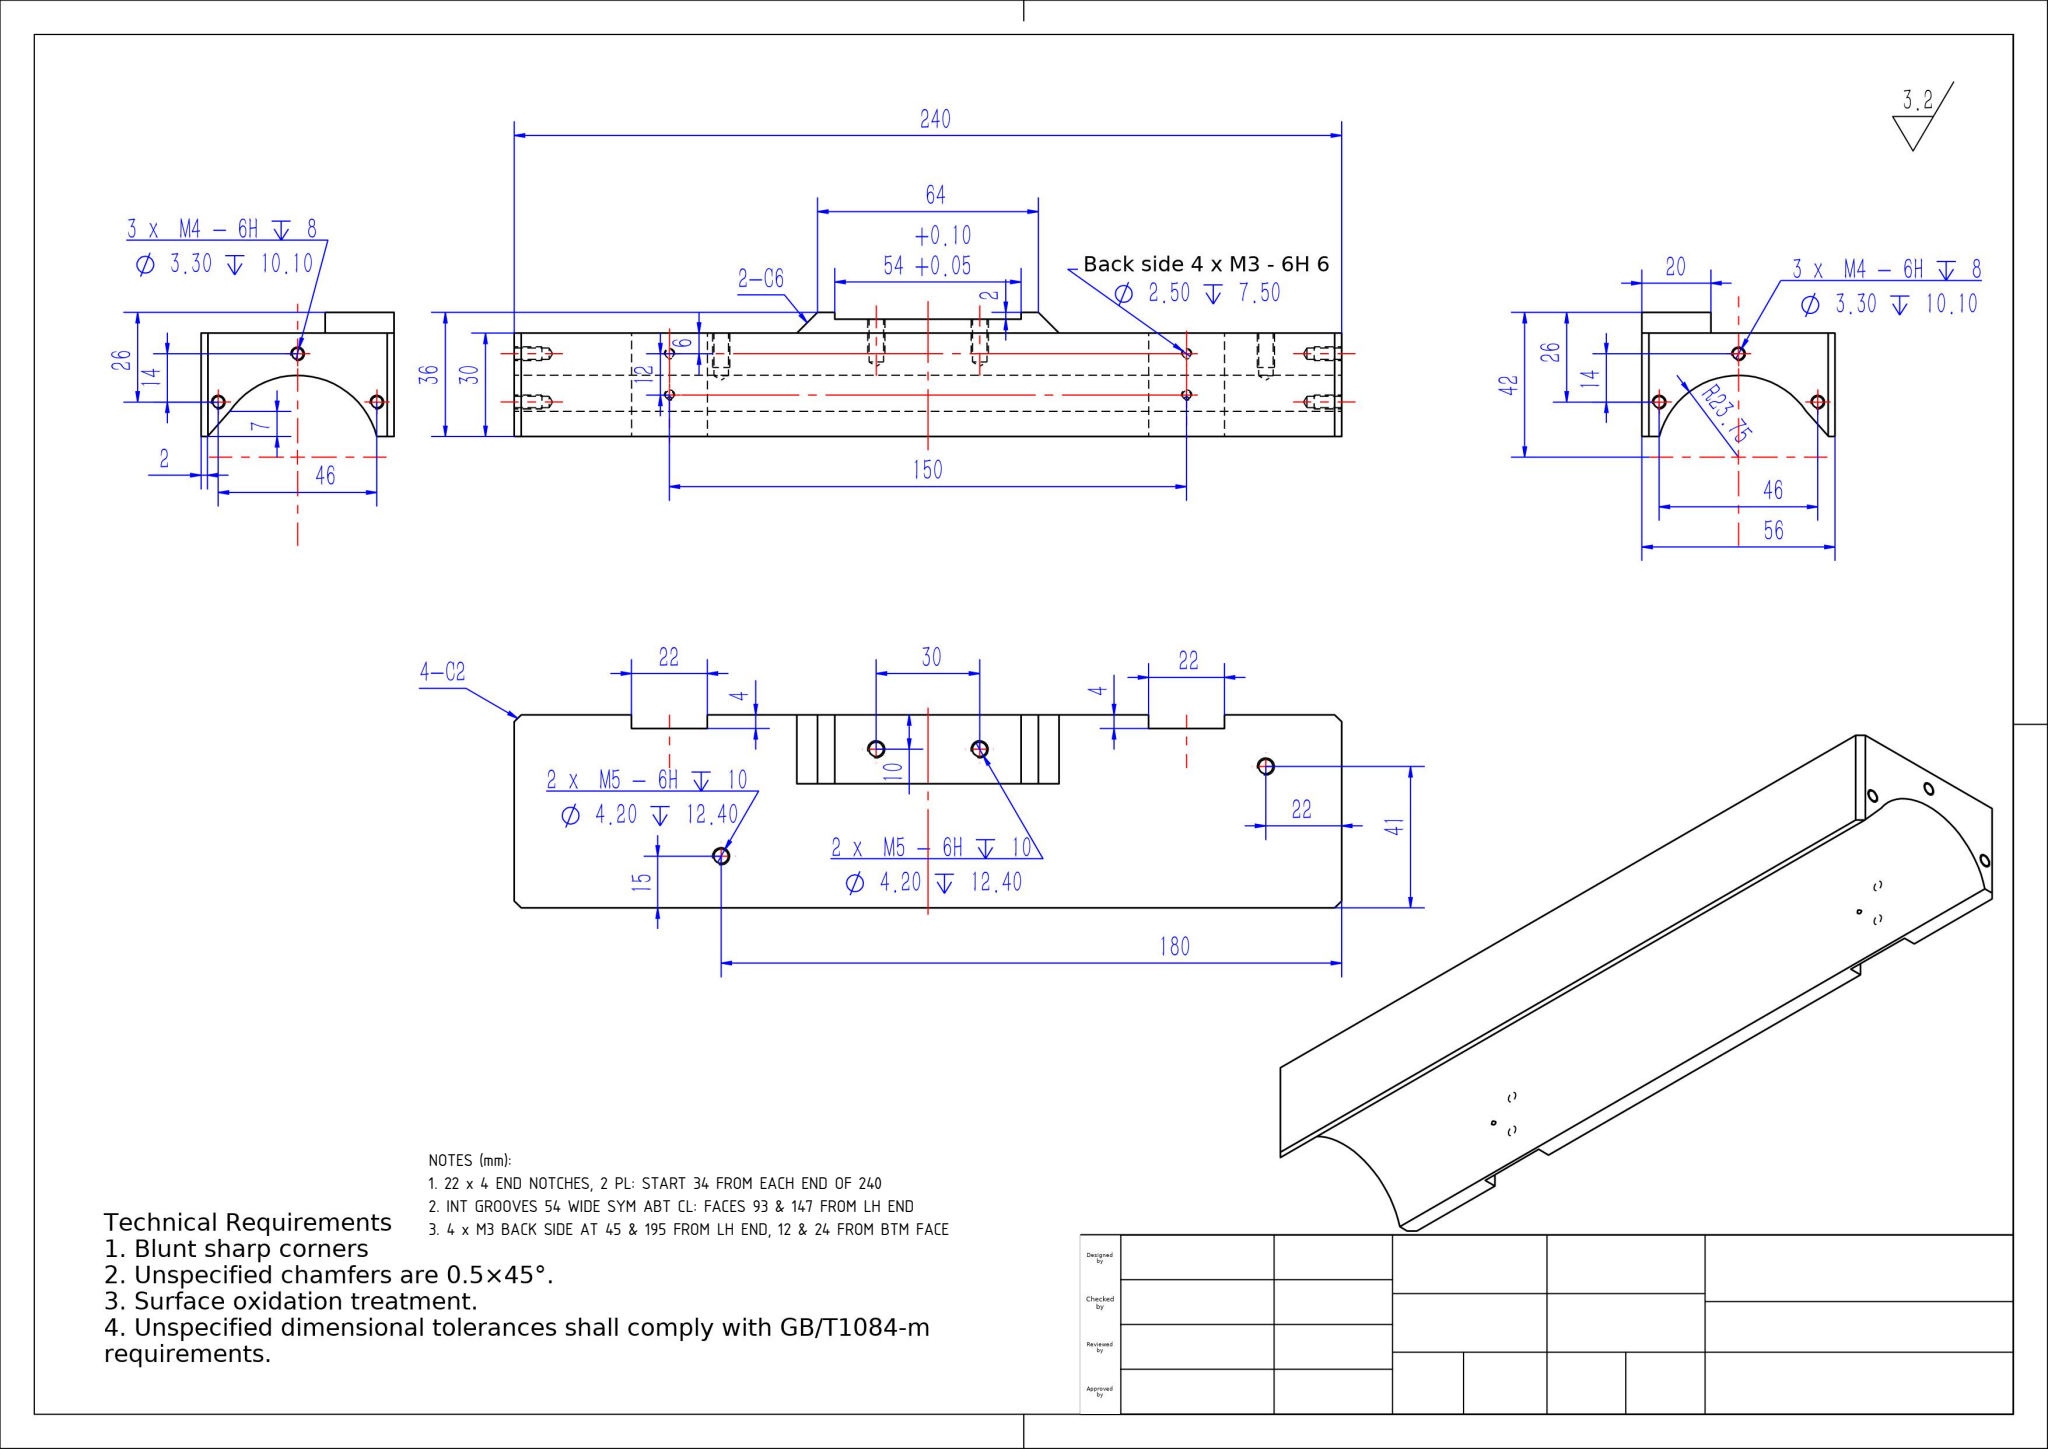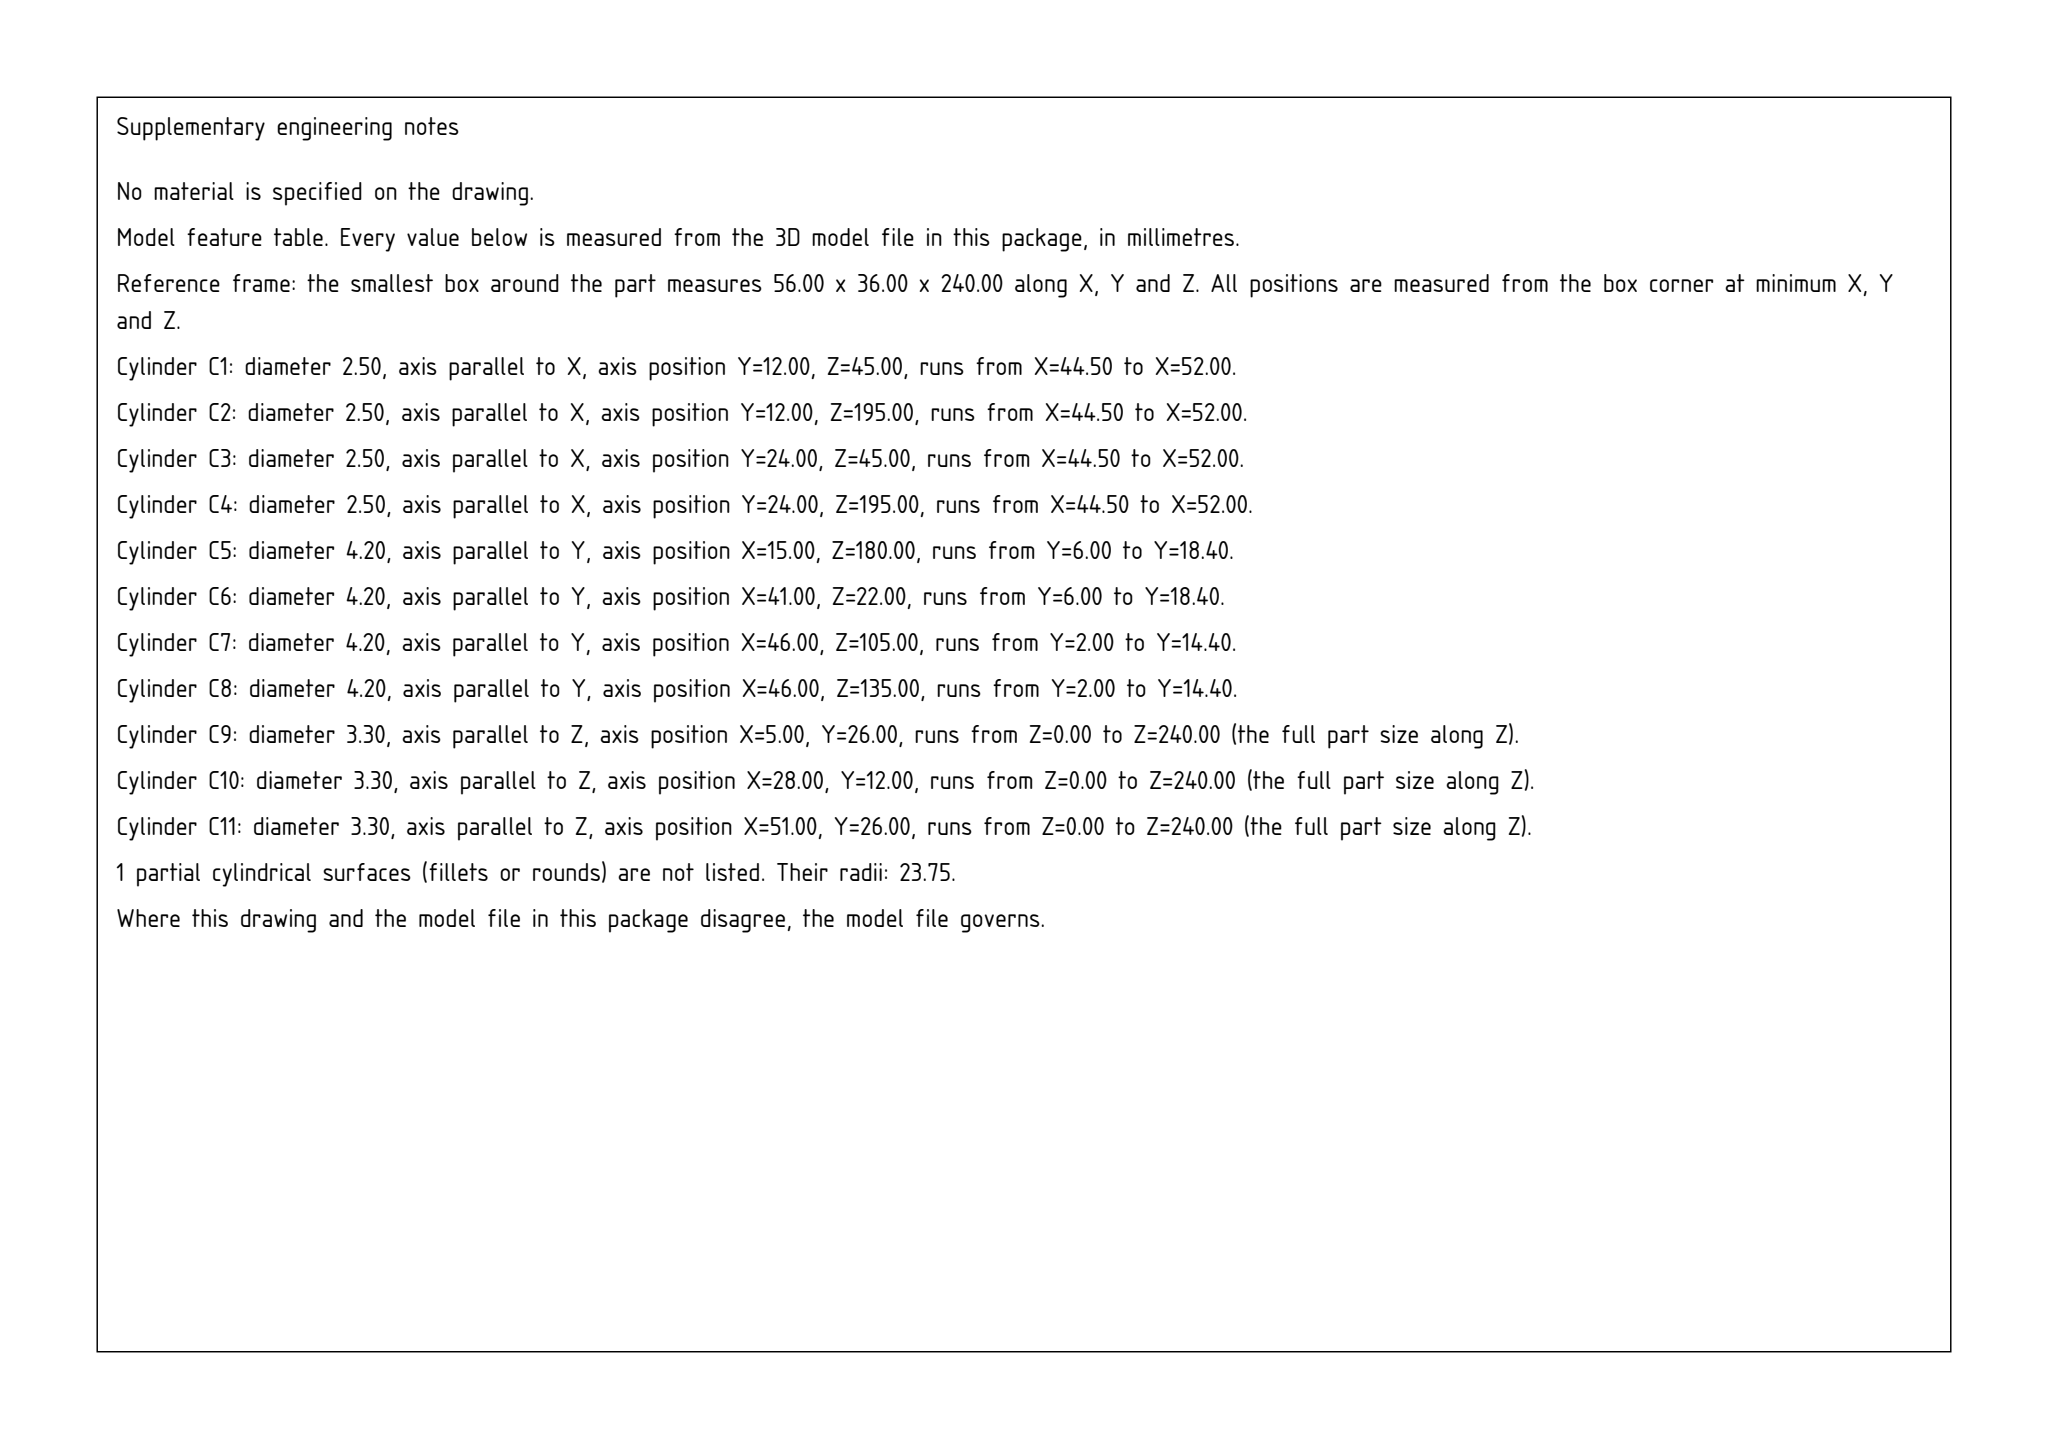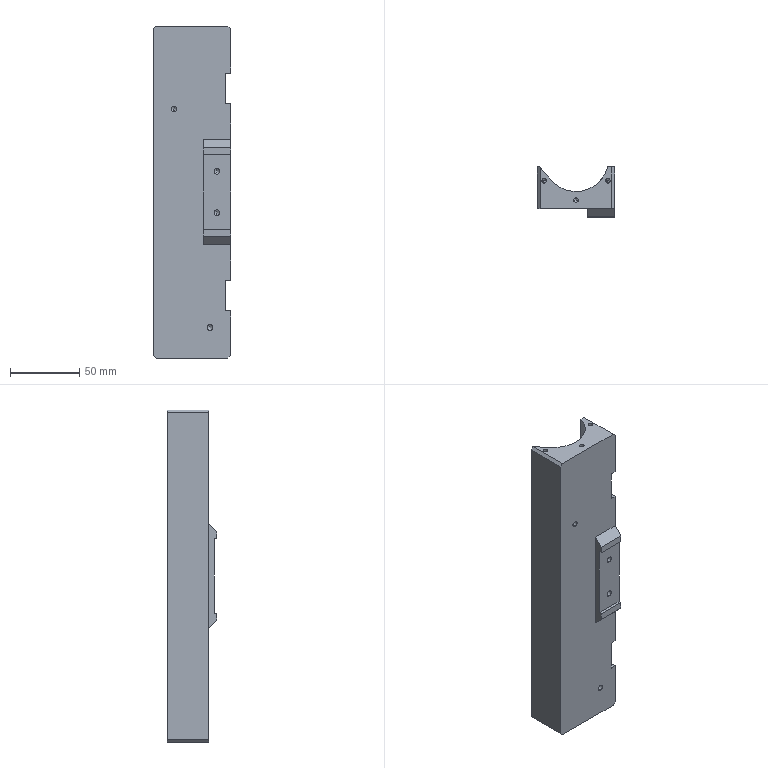Part | SolidWorks | mm | 1 solid | 85 faces | box 56 x 36 x 240 mm | volume 255219 mm3 | cylinder 29 | cone 28 | plane 28 | commonest cylinder face diameters 3.3 x12 4.2 x8 2.5 x8 47.5 x1
Drawing notes:
22 x 4 END NOTCHES, 2 PL: START 34 FROM EACH END OF 240 | from the solid: z planes 34/56 and 184/206 (22 lg); x planes 52 to 56 = 4 deep; 240-206=34
INT GROOVES 54 WIDE SYM ABT CL: FACES 93 & 147 FROM LH END | from the solid: z planes at 93 and 147, 54 apart, 93+147=240 so sym about mid-length
4 x M3 BACK SIDE AT 45 & 195 FROM LH END, 12 & 24 FROM BTM FACE | from the solid: Ø2.5 x-axis holes at (y12,z45),(y12,z195),(y24,z45),(y24,z195); 195-45=150